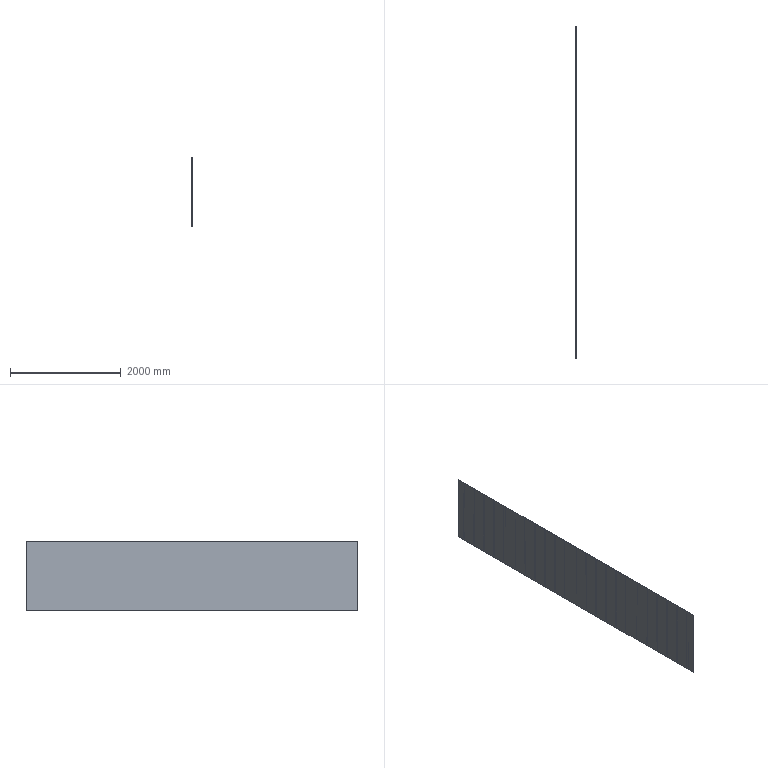Component | SolidWorks | Tread-63 | 1 solid | 121 faces | box 8 x 6000 x 1260 mm | volume 58846726 mm3 | plane 121
build123d program:
from build123d import *

# Parameters (mm, degrees)
SKETCH1_W               = 1260
SKETCH1_H               = 6000
BOSS_EXTRUDE1_DEPTH     = 8
SKETCH2_W               = 1183.532
SKETCH2_H               = 30
CUT_EXTRUDE_THIN1_DEPTH = 2
LPATTERN1_COUNT         = 23
LPATTERN1_PITCH         = 260


with BuildPart() as part:
    # Sketch1 → Boss-Extrude1 (new body)
    with BuildSketch(Plane.XY):
        with Locations((-5588.381, 10888.223)):
            Rectangle(SKETCH1_W, SKETCH1_H)
    extrude(amount=BOSS_EXTRUDE1_DEPTH)

    # Sketch2 → Cut-Extrude-Thin1 (cut)
    with BuildSketch(Plane(origin=(0, 0, 0), x_dir=(-1, 0, 0), z_dir=(0, 0, -1))):
        with Locations((5591.534, 8017.558)):
            Rectangle(SKETCH2_W, SKETCH2_H)
    cut_extrude_thin1 = extrude(amount=-CUT_EXTRUDE_THIN1_DEPTH, mode=Mode.SUBTRACT)

    # LPattern1: Cut-Extrude-Thin1 ×23
    with Locations(*[(0, i * LPATTERN1_PITCH, 0) for i in range(1, LPATTERN1_COUNT)]):
        add(cut_extrude_thin1, mode=Mode.SUBTRACT)


solid = part.part

# Placed as in the assembly
solid = solid.moved(Location((2077.926, 2768.376, -3539.381), (180, -90, 0)))